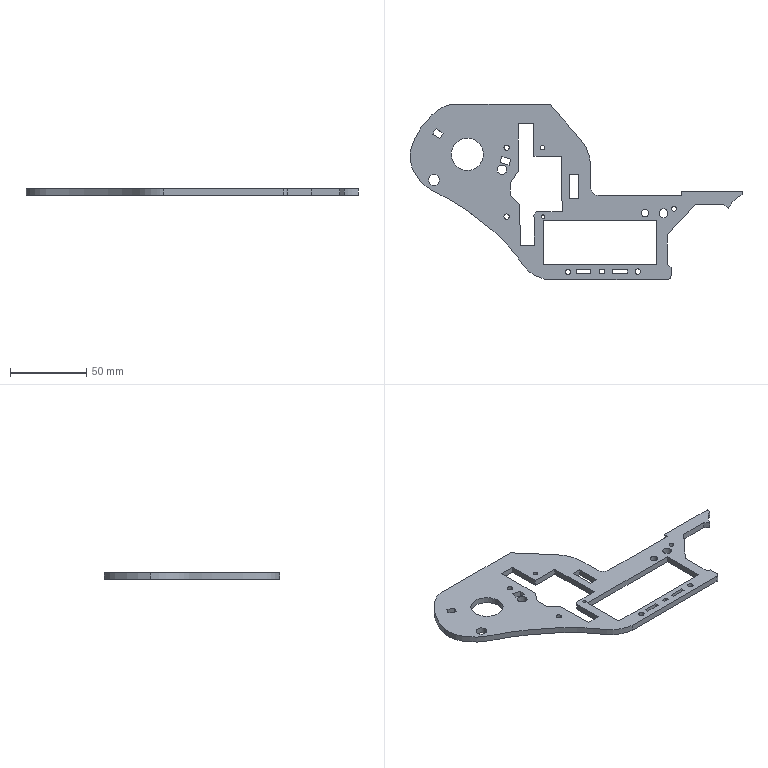Component | SolidWorks | MirrorSidePlate-2 | 1 solid | 88 faces | volume 34186 mm3 | plane 58 | cylinder 28 | spline 2 | commonest cylinder face diameters 3.467 x4 7.117 x2 21.091 x2 6.282 x2 3.459 x2 3.086 x2 4.983 x2 5.832 x2